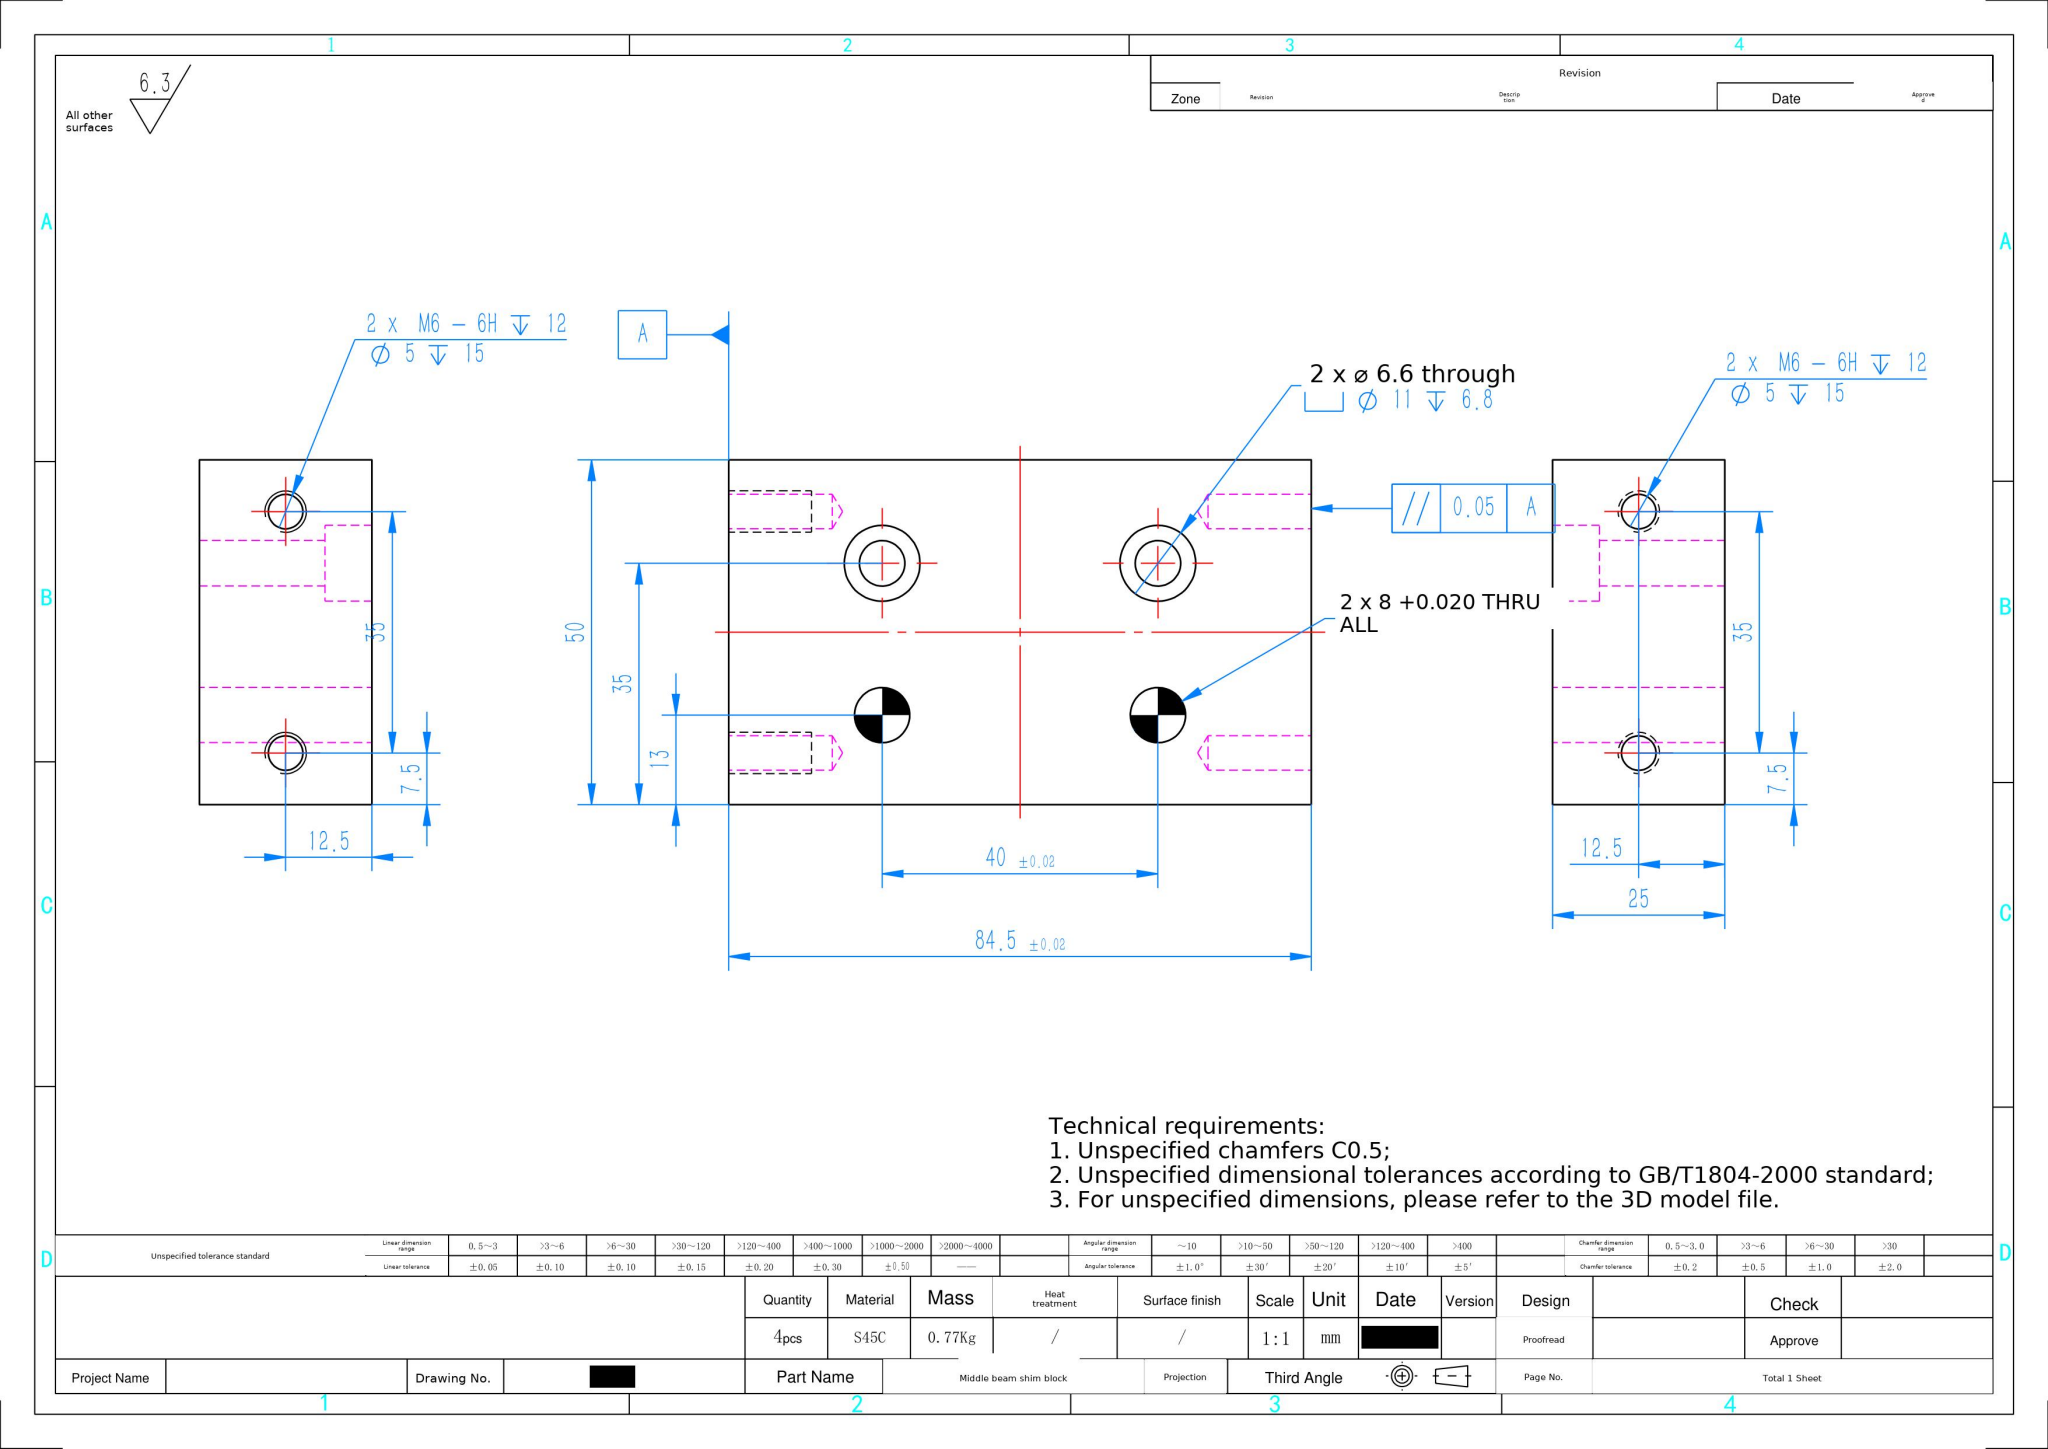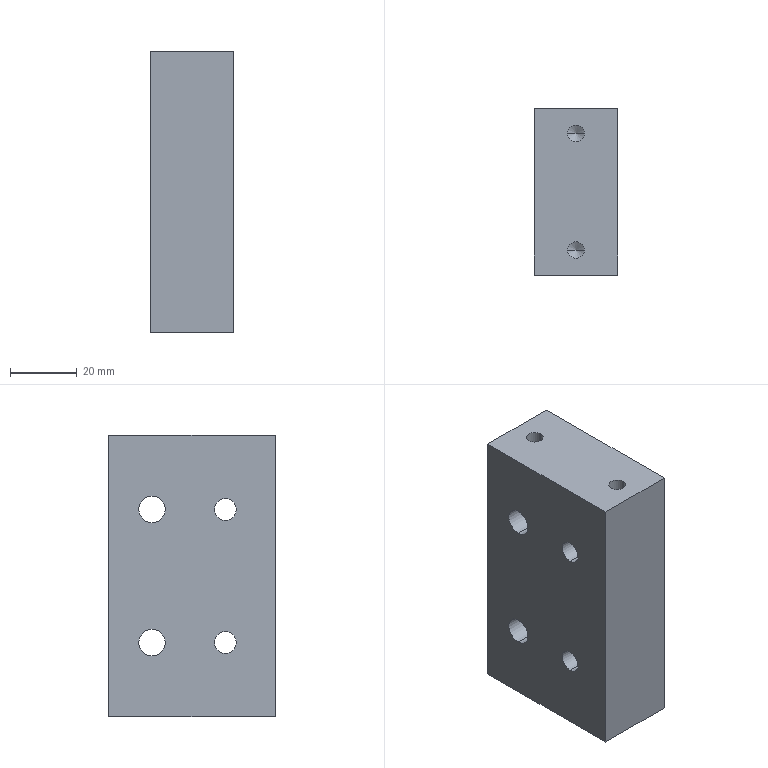Part | SolidWorks | mm | material S45C | 1 solid | 36 faces | box 25 x 50 x 84.5 mm | volume 99357 mm3 | cylinder 20 | cone 8 | plane 8 | commonest cylinder face diameters 5 x8 8 x4 11 x4 6.6 x4
STEP:
#1=CARTESIAN_POINT('',(10.,-17.5,27.25));
#2=VERTEX_POINT('',#1);
#3=CARTESIAN_POINT('',(15.,-17.5,27.25));
#4=VERTEX_POINT('',#3);
#5=CARTESIAN_POINT('',(12.5,-17.5,27.25));
#6=DIRECTION('',(0.,0.,1.));
#7=DIRECTION('',(1.,0.,0.));
#8=AXIS2_PLACEMENT_3D('',#5,#6,#7);
#9=CIRCLE('',#8,2.5);
#10=EDGE_CURVE('',#2,#4,#9,.T.);
#11=ORIENTED_EDGE('',*,*,#10,.F.);
#12=CARTESIAN_POINT('',(10.,-17.5,42.25));
#13=VERTEX_POINT('',#12);
#14=CARTESIAN_POINT('',(10.,-17.5,42.25));
#15=DIRECTION('',(0.,0.,1.));
#16=VECTOR('',#15,1000.);
#17=LINE('',#14,#16);
#18=EDGE_CURVE('',#2,#13,#17,.T.);
#19=ORIENTED_EDGE('',*,*,#18,.T.);
#20=CARTESIAN_POINT('',(15.,-17.5,42.25));
#21=VERTEX_POINT('',#20);
#22=CARTESIAN_POINT('',(12.5,-17.5,42.25));
#23=DIRECTION('',(0.,0.,1.));
#24=DIRECTION('',(1.,0.,0.));
#25=AXIS2_PLACEMENT_3D('',#22,#23,#24);
#26=CIRCLE('',#25,2.5);
#27=EDGE_CURVE('',#13,#21,#26,.T.);
#28=ORIENTED_EDGE('',*,*,#27,.T.);
#29=CARTESIAN_POINT('',(15.,-17.5,42.25));
#30=DIRECTION('',(0.,0.,1.));
#31=VECTOR('',#30,1000.);
#32=LINE('',#29,#31);
#33=EDGE_CURVE('',#4,#21,#32,.T.);
#34=ORIENTED_EDGE('',*,*,#33,.F.);
#35=EDGE_LOOP('',(#11,#19,#28,#34));
#36=FACE_OUTER_BOUND('',#35,.T.);
#37=CARTESIAN_POINT('',(12.5,-17.5,42.25));
#38=DIRECTION('',(0.,0.,1.));
#39=DIRECTION('',(1.,0.,0.));
#40=AXIS2_PLACEMENT_3D('',#37,#38,#39);
#41=CYLINDRICAL_SURFACE('',#40,2.5);
#42=ADVANCED_FACE('',(#36),#41,.F.);
#43=CARTESIAN_POINT('',(12.5,-17.5,25.748));
#44=VERTEX_POINT('',#43);
#45=CARTESIAN_POINT('',(15.,-17.5,27.25));
#46=DIRECTION('',(0.8572,0.,0.515));
#47=VECTOR('',#46,1000.);
#48=LINE('',#45,#47);
#49=EDGE_CURVE('',#44,#4,#48,.T.);
#50=ORIENTED_EDGE('',*,*,#49,.F.);
#51=CARTESIAN_POINT('',(10.,-17.5,27.25));
#52=DIRECTION('',(-0.8572,0.,0.515));
#53=VECTOR('',#52,1000.);
#54=LINE('',#51,#53);
#55=EDGE_CURVE('',#44,#2,#54,.T.);
#56=ORIENTED_EDGE('',*,*,#55,.T.);
#57=ORIENTED_EDGE('',*,*,#10,.T.);
#58=EDGE_LOOP('',(#50,#56,#57));
#59=FACE_OUTER_BOUND('',#58,.T.);
#60=CARTESIAN_POINT('',(12.5,-17.5,27.25));
#61=DIRECTION('',(0.,0.,1.));
#62=DIRECTION('',(1.,0.,0.));
#63=AXIS2_PLACEMENT_3D('',#60,#61,#62);
#64=CONICAL_SURFACE('',#63,2.5,1.03);
#65=ADVANCED_FACE('',(#59),#64,.F.);
#66=CARTESIAN_POINT('',(10.,17.5,27.25));
#67=VERTEX_POINT('',#66);
#68=CARTESIAN_POINT('',(15.,17.5,27.25));
#69=VERTEX_POINT('',#68);
#70=CARTESIAN_POINT('',(12.5,17.5,27.25));
#71=DIRECTION('',(0.,0.,1.));
#72=DIRECTION('',(1.,0.,0.));
#73=AXIS2_PLACEMENT_3D('',#70,#71,#72);
#74=CIRCLE('',#73,2.5);
#75=EDGE_CURVE('',#67,#69,#74,.T.);
#76=ORIENTED_EDGE('',*,*,#75,.F.);
#77=CARTESIAN_POINT('',(10.,17.5,42.25));
#78=VERTEX_POINT('',#77);
#79=CARTESIAN_POINT('',(10.,17.5,42.25));
#80=DIRECTION('',(0.,0.,1.));
#81=VECTOR('',#80,1000.);
#82=LINE('',#79,#81);
#83=EDGE_CURVE('',#67,#78,#82,.T.);
#84=ORIENTED_EDGE('',*,*,#83,.T.);
#85=CARTESIAN_POINT('',(15.,17.5,42.25));
#86=VERTEX_POINT('',#85);
#87=CARTESIAN_POINT('',(12.5,17.5,42.25));
#88=DIRECTION('',(0.,0.,1.));
#89=DIRECTION('',(1.,0.,0.));
#90=AXIS2_PLACEMENT_3D('',#87,#88,#89);
#91=CIRCLE('',#90,2.5);
#92=EDGE_CURVE('',#78,#86,#91,.T.);
#93=ORIENTED_EDGE('',*,*,#92,.T.);
#94=CARTESIAN_POINT('',(15.,17.5,42.25));
#95=DIRECTION('',(0.,0.,1.));
#96=VECTOR('',#95,1000.);
#97=LINE('',#94,#96);
#98=EDGE_CURVE('',#69,#86,#97,.T.);
#99=ORIENTED_EDGE('',*,*,#98,.F.);
#100=EDGE_LOOP('',(#76,#84,#93,#99));
#101=FACE_OUTER_BOUND('',#100,.T.);
#102=CARTESIAN_POINT('',(12.5,17.5,42.25));
#103=DIRECTION('',(0.,0.,1.));
#104=DIRECTION('',(1.,0.,0.));
#105=AXIS2_PLACEMENT_3D('',#102,#103,#104);
#106=CYLINDRICAL_SURFACE('',#105,2.5);
#107=ADVANCED_FACE('',(#101),#106,.F.);
#108=CARTESIAN_POINT('',(12.5,17.5,25.748));
#109=VERTEX_POINT('',#108);
#110=CARTESIAN_POINT('',(15.,17.5,27.25));
#111=DIRECTION('',(0.8572,0.,0.515));
#112=VECTOR('',#111,1000.);
#113=LINE('',#110,#112);
#114=EDGE_CURVE('',#109,#69,#113,.T.);
#115=ORIENTED_EDGE('',*,*,#114,.F.);
#116=CARTESIAN_POINT('',(10.,17.5,27.25));
#117=DIRECTION('',(-0.8572,0.,0.515));
#118=VECTOR('',#117,1000.);
#119=LINE('',#116,#118);
#120=EDGE_CURVE('',#109,#67,#119,.T.);
#121=ORIENTED_EDGE('',*,*,#120,.T.);
#122=ORIENTED_EDGE('',*,*,#75,.T.);
#123=EDGE_LOOP('',(#115,#121,#122));
#124=FACE_OUTER_BOUND('',#123,.T.);
#125=CARTESIAN_POINT('',(12.5,17.5,27.25));
#126=DIRECTION('',(0.,0.,1.));
#127=DIRECTION('',(1.,0.,0.));
#128=AXIS2_PLACEMENT_3D('',#125,#126,#127);
#129=CONICAL_SURFACE('',#128,2.5,1.03);
#130=ADVANCED_FACE('',(#124),#129,.F.);
#131=CARTESIAN_POINT('',(15.,17.5,-27.25));
#132=VERTEX_POINT('',#131);
#133=CARTESIAN_POINT('',(10.,17.5,-27.25));
#134=VERTEX_POINT('',#133);
#135=CARTESIAN_POINT('',(12.5,17.5,-27.25));
#136=DIRECTION('',(0.,0.,-1.));
#137=DIRECTION('',(-1.,0.,0.));
#138=AXIS2_PLACEMENT_3D('',#135,#136,#137);
#139=CIRCLE('',#138,2.5);
#140=EDGE_CURVE('',#132,#134,#139,.T.);
#141=ORIENTED_EDGE('',*,*,#140,.F.);
#142=CARTESIAN_POINT('',(15.,17.5,-42.25));
#143=VERTEX_POINT('',#142);
#144=CARTESIAN_POINT('',(15.,17.5,-42.25));
#145=DIRECTION('',(0.,0.,-1.));
#146=VECTOR('',#145,1000.);
#147=LINE('',#144,#146);
#148=EDGE_CURVE('',#132,#143,#147,.T.);
#149=ORIENTED_EDGE('',*,*,#148,.T.);
#150=CARTESIAN_POINT('',(10.,17.5,-42.25));
#151=VERTEX_POINT('',#150);
#152=CARTESIAN_POINT('',(12.5,17.5,-42.25));
#153=DIRECTION('',(0.,0.,-1.));
#154=DIRECTION('',(-1.,0.,0.));
#155=AXIS2_PLACEMENT_3D('',#152,#153,#154);
#156=CIRCLE('',#155,2.5);
#157=EDGE_CURVE('',#143,#151,#156,.T.);
#158=ORIENTED_EDGE('',*,*,#157,.T.);
#159=CARTESIAN_POINT('',(10.,17.5,-42.25));
#160=DIRECTION('',(0.,0.,-1.));
#161=VECTOR('',#160,1000.);
#162=LINE('',#159,#161);
#163=EDGE_CURVE('',#134,#151,#162,.T.);
#164=ORIENTED_EDGE('',*,*,#163,.F.);
#165=EDGE_LOOP('',(#141,#149,#158,#164));
#166=FACE_OUTER_BOUND('',#165,.T.);
#167=CARTESIAN_POINT('',(12.5,17.5,-42.25));
#168=DIRECTION('',(0.,0.,-1.));
#169=DIRECTION('',(-1.,0.,0.));
#170=AXIS2_PLACEMENT_3D('',#167,#168,#169);
#171=CYLINDRICAL_SURFACE('',#170,2.5);
#172=ADVANCED_FACE('',(#166),#171,.F.);
#173=CARTESIAN_POINT('',(12.5,17.5,-25.748));
#174=VERTEX_POINT('',#173);
#175=CARTESIAN_POINT('',(10.,17.5,-27.25));
#176=DIRECTION('',(-0.8572,0.,-0.515));
#177=VECTOR('',#176,1000.);
#178=LINE('',#175,#177);
#179=EDGE_CURVE('',#174,#134,#178,.T.);
#180=ORIENTED_EDGE('',*,*,#179,.F.);
#181=CARTESIAN_POINT('',(15.,17.5,-27.25));
#182=DIRECTION('',(0.8572,0.,-0.515));
#183=VECTOR('',#182,1000.);
#184=LINE('',#181,#183);
#185=EDGE_CURVE('',#174,#132,#184,.T.);
#186=ORIENTED_EDGE('',*,*,#185,.T.);
#187=ORIENTED_EDGE('',*,*,#140,.T.);
#188=EDGE_LOOP('',(#180,#186,#187));
#189=FACE_OUTER_BOUND('',#188,.T.);
#190=CARTESIAN_POINT('',(12.5,17.5,-27.25));
#191=DIRECTION('',(0.,0.,-1.));
#192=DIRECTION('',(-1.,0.,0.));
#193=AXIS2_PLACEMENT_3D('',#190,#191,#192);
#194=CONICAL_SURFACE('',#193,2.5,1.03);
#195=ADVANCED_FACE('',(#189),#194,.F.);
#196=CARTESIAN_POINT('',(15.,-17.5,-27.25));
#197=VERTEX_POINT('',#196);
#198=CARTESIAN_POINT('',(10.,-17.5,-27.25));
#199=VERTEX_POINT('',#198);
#200=CARTESIAN_POINT('',(12.5,-17.5,-27.25));
#201=DIRECTION('',(0.,0.,-1.));
#202=DIRECTION('',(-1.,0.,0.));
#203=AXIS2_PLACEMENT_3D('',#200,#201,#202);
#204=CIRCLE('',#203,2.5);
#205=EDGE_CURVE('',#197,#199,#204,.T.);
#206=ORIENTED_EDGE('',*,*,#205,.F.);
#207=CARTESIAN_POINT('',(15.,-17.5,-42.25));
#208=VERTEX_POINT('',#207);
#209=CARTESIAN_POINT('',(15.,-17.5,-42.25));
#210=DIRECTION('',(0.,0.,-1.));
#211=VECTOR('',#210,1000.);
#212=LINE('',#209,#211);
#213=EDGE_CURVE('',#197,#208,#212,.T.);
#214=ORIENTED_EDGE('',*,*,#213,.T.);
#215=CARTESIAN_POINT('',(10.,-17.5,-42.25));
#216=VERTEX_POINT('',#215);
#217=CARTESIAN_POINT('',(12.5,-17.5,-42.25));
#218=DIRECTION('',(0.,0.,-1.));
#219=DIRECTION('',(-1.,0.,0.));
#220=AXIS2_PLACEMENT_3D('',#217,#218,#219);
#221=CIRCLE('',#220,2.5);
#222=EDGE_CURVE('',#208,#216,#221,.T.);
#223=ORIENTED_EDGE('',*,*,#222,.T.);
#224=CARTESIAN_POINT('',(10.,-17.5,-42.25));
#225=DIRECTION('',(0.,0.,-1.));
#226=VECTOR('',#225,1000.);
#227=LINE('',#224,#226);
#228=EDGE_CURVE('',#199,#216,#227,.T.);
#229=ORIENTED_EDGE('',*,*,#228,.F.);
#230=EDGE_LOOP('',(#206,#214,#223,#229));
#231=FACE_OUTER_BOUND('',#230,.T.);
#232=CARTESIAN_POINT('',(12.5,-17.5,-42.25));
#233=DIRECTION('',(0.,0.,-1.));
#234=DIRECTION('',(-1.,0.,0.));
#235=AXIS2_PLACEMENT_3D('',#232,#233,#234);
#236=CYLINDRICAL_SURFACE('',#235,2.5);
#237=ADVANCED_FACE('',(#231),#236,.F.);
#238=CARTESIAN_POINT('',(12.5,-17.5,-25.748));
#239=VERTEX_POINT('',#238);
#240=CARTESIAN_POINT('',(10.,-17.5,-27.25));
#241=DIRECTION('',(-0.8572,0.,-0.515));
#242=VECTOR('',#241,1000.);
#243=LINE('',#240,#242);
#244=EDGE_CURVE('',#239,#199,#243,.T.);
#245=ORIENTED_EDGE('',*,*,#244,.F.);
#246=CARTESIAN_POINT('',(15.,-17.5,-27.25));
#247=DIRECTION('',(0.8572,0.,-0.515));
#248=VECTOR('',#247,1000.);
#249=LINE('',#246,#248);
#250=EDGE_CURVE('',#239,#197,#249,.T.);
#251=ORIENTED_EDGE('',*,*,#250,.T.);
#252=ORIENTED_EDGE('',*,*,#205,.T.);
#253=EDGE_LOOP('',(#245,#251,#252));
#254=FACE_OUTER_BOUND('',#253,.T.);
#255=CARTESIAN_POINT('',(12.5,-17.5,-27.25));
#256=DIRECTION('',(0.,0.,-1.));
#257=DIRECTION('',(-1.,0.,0.));
#258=AXIS2_PLACEMENT_3D('',#255,#256,#257);
#259=CONICAL_SURFACE('',#258,2.5,1.03);
#260=ADVANCED_FACE('',(#254),#259,.F.);
#261=CARTESIAN_POINT('',(0.,12.,-16.));
#262=VERTEX_POINT('',#261);
#263=CARTESIAN_POINT('',(0.,12.,-24.));
#264=VERTEX_POINT('',#263);
#265=CARTESIAN_POINT('',(0.,12.,-20.));
#266=DIRECTION('',(1.,0.,0.));
#267=DIRECTION('',(0.,0.,-1.));
#268=AXIS2_PLACEMENT_3D('',#265,#266,#267);
#269=CIRCLE('',#268,4.);
#270=EDGE_CURVE('',#262,#264,#269,.T.);
#271=ORIENTED_EDGE('',*,*,#270,.F.);
#272=CARTESIAN_POINT('',(25.,12.,-16.));
#273=VERTEX_POINT('',#272);
#274=CARTESIAN_POINT('',(25.,12.,-16.));
#275=DIRECTION('',(1.,0.,0.));
#276=VECTOR('',#275,1000.);
#277=LINE('',#274,#276);
#278=EDGE_CURVE('',#262,#273,#277,.T.);
#279=ORIENTED_EDGE('',*,*,#278,.T.);
#280=CARTESIAN_POINT('',(25.,12.,-24.));
#281=VERTEX_POINT('',#280);
#282=CARTESIAN_POINT('',(25.,12.,-20.));
#283=DIRECTION('',(1.,0.,0.));
#284=DIRECTION('',(0.,0.,-1.));
#285=AXIS2_PLACEMENT_3D('',#282,#283,#284);
#286=CIRCLE('',#285,4.);
#287=EDGE_CURVE('',#273,#281,#286,.T.);
#288=ORIENTED_EDGE('',*,*,#287,.T.);
#289=CARTESIAN_POINT('',(25.,12.,-24.));
#290=DIRECTION('',(1.,0.,0.));
#291=VECTOR('',#290,1000.);
#292=LINE('',#289,#291);
#293=EDGE_CURVE('',#264,#281,#292,.T.);
#294=ORIENTED_EDGE('',*,*,#293,.F.);
#295=EDGE_LOOP('',(#271,#279,#288,#294));
#296=FACE_OUTER_BOUND('',#295,.T.);
#297=CARTESIAN_POINT('',(25.,12.,-20.));
#298=DIRECTION('',(1.,0.,0.));
#299=DIRECTION('',(0.,0.,-1.));
#300=AXIS2_PLACEMENT_3D('',#297,#298,#299);
#301=CYLINDRICAL_SURFACE('',#300,4.);
#302=ADVANCED_FACE('',(#296),#301,.F.);
#303=CARTESIAN_POINT('',(0.,12.,24.));
#304=VERTEX_POINT('',#303);
#305=CARTESIAN_POINT('',(0.,12.,16.));
#306=VERTEX_POINT('',#305);
#307=CARTESIAN_POINT('',(0.,12.,20.));
#308=DIRECTION('',(1.,0.,0.));
#309=DIRECTION('',(0.,0.,-1.));
#310=AXIS2_PLACEMENT_3D('',#307,#308,#309);
#311=CIRCLE('',#310,4.);
#312=EDGE_CURVE('',#304,#306,#311,.T.);
#313=ORIENTED_EDGE('',*,*,#312,.F.);
#314=CARTESIAN_POINT('',(25.,12.,24.));
#315=VERTEX_POINT('',#314);
#316=CARTESIAN_POINT('',(25.,12.,24.));
#317=DIRECTION('',(1.,0.,0.));
#318=VECTOR('',#317,1000.);
#319=LINE('',#316,#318);
#320=EDGE_CURVE('',#304,#315,#319,.T.);
#321=ORIENTED_EDGE('',*,*,#320,.T.);
#322=CARTESIAN_POINT('',(25.,12.,16.));
#323=VERTEX_POINT('',#322);
#324=CARTESIAN_POINT('',(25.,12.,20.));
#325=DIRECTION('',(1.,0.,0.));
#326=DIRECTION('',(0.,0.,-1.));
#327=AXIS2_PLACEMENT_3D('',#324,#325,#326);
#328=CIRCLE('',#327,4.);
#329=EDGE_CURVE('',#315,#323,#328,.T.);
#330=ORIENTED_EDGE('',*,*,#329,.T.);
#331=CARTESIAN_POINT('',(25.,12.,16.));
#332=DIRECTION('',(1.,0.,0.));
#333=VECTOR('',#332,1000.);
#334=LINE('',#331,#333);
#335=EDGE_CURVE('',#306,#323,#334,.T.);
#336=ORIENTED_EDGE('',*,*,#335,.F.);
#337=EDGE_LOOP('',(#313,#321,#330,#336));
#338=FACE_OUTER_BOUND('',#337,.T.);
#339=CARTESIAN_POINT('',(25.,12.,20.));
#340=DIRECTION('',(1.,0.,0.));
#341=DIRECTION('',(0.,0.,-1.));
#342=AXIS2_PLACEMENT_3D('',#339,#340,#341);
#343=CYLINDRICAL_SURFACE('',#342,4.);
#344=ADVANCED_FACE('',(#338),#343,.F.);
#345=CARTESIAN_POINT('',(18.2,-10.,-14.5));
#346=VERTEX_POINT('',#345);
#347=CARTESIAN_POINT('',(18.2,-10.,-25.5));
#348=VERTEX_POINT('',#347);
#349=CARTESIAN_POINT('',(18.2,-10.,-20.));
#350=DIRECTION('',(1.,0.,0.));
#351=DIRECTION('',(0.,0.,-1.));
#352=AXIS2_PLACEMENT_3D('',#349,#350,#351);
#353=CIRCLE('',#352,5.5);
#354=EDGE_CURVE('',#346,#348,#353,.T.);
#355=ORIENTED_EDGE('',*,*,#354,.F.);
#356=CARTESIAN_POINT('',(25.,-10.,-14.5));
#357=VERTEX_POINT('',#356);
#358=CARTESIAN_POINT('',(25.,-10.,-14.5));
#359=DIRECTION('',(1.,0.,0.));
#360=VECTOR('',#359,1000.);
#361=LINE('',#358,#360);
#362=EDGE_CURVE('',#346,#357,#361,.T.);
#363=ORIENTED_EDGE('',*,*,#362,.T.);
#364=CARTESIAN_POINT('',(25.,-10.,-25.5));
#365=VERTEX_POINT('',#364);
#366=CARTESIAN_POINT('',(25.,-10.,-20.));
#367=DIRECTION('',(1.,0.,0.));
#368=DIRECTION('',(0.,0.,-1.));
#369=AXIS2_PLACEMENT_3D('',#366,#367,#368);
#370=CIRCLE('',#369,5.5);
#371=EDGE_CURVE('',#357,#365,#370,.T.);
#372=ORIENTED_EDGE('',*,*,#371,.T.);
#373=CARTESIAN_POINT('',(25.,-10.,-25.5));
#374=DIRECTION('',(1.,0.,0.));
#375=VECTOR('',#374,1000.);
#376=LINE('',#373,#375);
#377=EDGE_CURVE('',#348,#365,#376,.T.);
#378=ORIENTED_EDGE('',*,*,#377,.F.);
#379=EDGE_LOOP('',(#355,#363,#372,#378));
#380=FACE_OUTER_BOUND('',#379,.T.);
#381=CARTESIAN_POINT('',(25.,-10.,-20.));
#382=DIRECTION('',(1.,0.,0.));
#383=DIRECTION('',(0.,0.,-1.));
#384=AXIS2_PLACEMENT_3D('',#381,#382,#383);
#385=CYLINDRICAL_SURFACE('',#384,5.5);
#386=ADVANCED_FACE('',(#380),#385,.F.);
#387=CARTESIAN_POINT('',(0.,-10.,-16.7));
#388=VERTEX_POINT('',#387);
#389=CARTESIAN_POINT('',(0.,-10.,-23.3));
#390=VERTEX_POINT('',#389);
#391=CARTESIAN_POINT('',(0.,-10.,-20.));
#392=DIRECTION('',(1.,0.,0.));
#393=DIRECTION('',(0.,0.,-1.));
#394=AXIS2_PLACEMENT_3D('',#391,#392,#393);
#395=CIRCLE('',#394,3.3);
#396=EDGE_CURVE('',#388,#390,#395,.T.);
#397=ORIENTED_EDGE('',*,*,#396,.F.);
#398=CARTESIAN_POINT('',(18.2,-10.,-16.7));
#399=VERTEX_POINT('',#398);
#400=CARTESIAN_POINT('',(25.,-10.,-16.7));
#401=DIRECTION('',(1.,0.,0.));
#402=VECTOR('',#401,1000.);
#403=LINE('',#400,#402);
#404=EDGE_CURVE('',#388,#399,#403,.T.);
#405=ORIENTED_EDGE('',*,*,#404,.T.);
#406=CARTESIAN_POINT('',(18.2,-10.,-23.3));
#407=VERTEX_POINT('',#406);
#408=CARTESIAN_POINT('',(18.2,-10.,-20.));
#409=DIRECTION('',(1.,0.,0.));
#410=DIRECTION('',(0.,0.,-1.));
#411=AXIS2_PLACEMENT_3D('',#408,#409,#410);
#412=CIRCLE('',#411,3.3);
#413=EDGE_CURVE('',#399,#407,#412,.T.);
#414=ORIENTED_EDGE('',*,*,#413,.T.);
#415=CARTESIAN_POINT('',(25.,-10.,-23.3));
#416=DIRECTION('',(1.,0.,0.));
#417=VECTOR('',#416,1000.);
#418=LINE('',#415,#417);
#419=EDGE_CURVE('',#390,#407,#418,.T.);
#420=ORIENTED_EDGE('',*,*,#419,.F.);
#421=EDGE_LOOP('',(#397,#405,#414,#420));
#422=FACE_OUTER_BOUND('',#421,.T.);
#423=CARTESIAN_POINT('',(25.,-10.,-20.));
#424=DIRECTION('',(1.,0.,0.));
#425=DIRECTION('',(0.,0.,-1.));
#426=AXIS2_PLACEMENT_3D('',#423,#424,#425);
#427=CYLINDRICAL_SURFACE('',#426,3.3);
#428=ADVANCED_FACE('',(#422),#427,.F.);
#429=CARTESIAN_POINT('',(18.2,-10.,25.5));
#430=VERTEX_POINT('',#429);
#431=CARTESIAN_POINT('',(18.2,-10.,14.5));
#432=VERTEX_POINT('',#431);
#433=CARTESIAN_POINT('',(18.2,-10.,20.));
#434=DIRECTION('',(1.,0.,0.));
#435=DIRECTION('',(0.,0.,-1.));
#436=AXIS2_PLACEMENT_3D('',#433,#434,#435);
#437=CIRCLE('',#436,5.5);
#438=EDGE_CURVE('',#430,#432,#437,.T.);
#439=ORIENTED_EDGE('',*,*,#438,.F.);
#440=CARTESIAN_POINT('',(25.,-10.,25.5));
#441=VERTEX_POINT('',#440);
#442=CARTESIAN_POINT('',(25.,-10.,25.5));
#443=DIRECTION('',(1.,0.,0.));
#444=VECTOR('',#443,1000.);
#445=LINE('',#442,#444);
#446=EDGE_CURVE('',#430,#441,#445,.T.);
#447=ORIENTED_EDGE('',*,*,#446,.T.);
#448=CARTESIAN_POINT('',(25.,-10.,14.5));
#449=VERTEX_POINT('',#448);
#450=CARTESIAN_POINT('',(25.,-10.,20.));
#451=DIRECTION('',(1.,0.,0.));
#452=DIRECTION('',(0.,0.,-1.));
#453=AXIS2_PLACEMENT_3D('',#450,#451,#452);
#454=CIRCLE('',#453,5.5);
#455=EDGE_CURVE('',#441,#449,#454,.T.);
#456=ORIENTED_EDGE('',*,*,#455,.T.);
#457=CARTESIAN_POINT('',(25.,-10.,14.5));
#458=DIRECTION('',(1.,0.,0.));
#459=VECTOR('',#458,1000.);
#460=LINE('',#457,#459);
#461=EDGE_CURVE('',#432,#449,#460,.T.);
#462=ORIENTED_EDGE('',*,*,#461,.F.);
#463=EDGE_LOOP('',(#439,#447,#456,#462));
#464=FACE_OUTER_BOUND('',#463,.T.);
#465=CARTESIAN_POINT('',(25.,-10.,20.));
#466=DIRECTION('',(1.,0.,0.));
#467=DIRECTION('',(0.,0.,-1.));
#468=AXIS2_PLACEMENT_3D('',#465,#466,#467);
#469=CYLINDRICAL_SURFACE('',#468,5.5);
#470=ADVANCED_FACE('',(#464),#469,.F.);
#471=CARTESIAN_POINT('',(0.,-10.,23.3));
#472=VERTEX_POINT('',#471);
#473=CARTESIAN_POINT('',(0.,-10.,16.7));
#474=VERTEX_POINT('',#473);
#475=CARTESIAN_POINT('',(0.,-10.,20.));
#476=DIRECTION('',(1.,0.,0.));
#477=DIRECTION('',(0.,0.,-1.));
#478=AXIS2_PLACEMENT_3D('',#475,#476,#477);
#479=CIRCLE('',#478,3.3);
#480=EDGE_CURVE('',#472,#474,#479,.T.);
#481=ORIENTED_EDGE('',*,*,#480,.F.);
#482=CARTESIAN_POINT('',(18.2,-10.,23.3));
#483=VERTEX_POINT('',#482);
#484=CARTESIAN_POINT('',(25.,-10.,23.3));
#485=DIRECTION('',(1.,0.,0.));
#486=VECTOR('',#485,1000.);
#487=LINE('',#484,#486);
#488=EDGE_CURVE('',#472,#483,#487,.T.);
#489=ORIENTED_EDGE('',*,*,#488,.T.);
#490=CARTESIAN_POINT('',(18.2,-10.,16.7));
#491=VERTEX_POINT('',#490);
#492=CARTESIAN_POINT('',(18.2,-10.,20.));
#493=DIRECTION('',(1.,0.,0.));
#494=DIRECTION('',(0.,0.,-1.));
#495=AXIS2_PLACEMENT_3D('',#492,#493,#494);
#496=CIRCLE('',#495,3.3);
#497=EDGE_CURVE('',#483,#491,#496,.T.);
#498=ORIENTED_EDGE('',*,*,#497,.T.);
#499=CARTESIAN_POINT('',(25.,-10.,16.7));
#500=DIRECTION('',(1.,0.,0.));
#501=VECTOR('',#500,1000.);
#502=LINE('',#499,#501);
#503=EDGE_CURVE('',#474,#491,#502,.T.);
#504=ORIENTED_EDGE('',*,*,#503,.F.);
#505=EDGE_LOOP('',(#481,#489,#498,#504));
#506=FACE_OUTER_BOUND('',#505,.T.);
#507=CARTESIAN_POINT('',(25.,-10.,20.));
#508=DIRECTION('',(1.,0.,0.));
#509=DIRECTION('',(0.,0.,-1.));
#510=AXIS2_PLACEMENT_3D('',#507,#508,#509);
#511=CYLINDRICAL_SURFACE('',#510,3.3);
#512=ADVANCED_FACE('',(#506),#511,.F.);
#513=CARTESIAN_POINT('',(12.5,17.5,-42.25));
#514=DIRECTION('',(0.,0.,-1.));
#515=DIRECTION('',(-1.,0.,0.));
#516=AXIS2_PLACEMENT_3D('',#513,#514,#515);
#517=CIRCLE('',#516,2.5);
#518=EDGE_CURVE('',#151,#143,#517,.T.);
#519=ORIENTED_EDGE('',*,*,#518,.F.);
#520=ORIENTED_EDGE('',*,*,#157,.F.);
#521=EDGE_LOOP('',(#519,#520));
#522=FACE_BOUND('',#521,.T.);
#523=CARTESIAN_POINT('',(12.5,-17.5,-42.25));
#524=DIRECTION('',(0.,0.,-1.));
#525=DIRECTION('',(-1.,0.,0.));
#526=AXIS2_PLACEMENT_3D('',#523,#524,#525);
#527=CIRCLE('',#526,2.5);
#528=EDGE_CURVE('',#216,#208,#527,.T.);
#529=ORIENTED_EDGE('',*,*,#528,.F.);
#530=ORIENTED_EDGE('',*,*,#222,.F.);
#531=EDGE_LOOP('',(#529,#530));
#532=FACE_BOUND('',#531,.T.);
#533=CARTESIAN_POINT('',(0.,-25.,-42.25));
#534=VERTEX_POINT('',#533);
#535=CARTESIAN_POINT('',(0.,25.,-42.25));
#536=VERTEX_POINT('',#535);
#537=CARTESIAN_POINT('',(0.,25.,-42.25));
#538=DIRECTION('',(0.,1.,0.));
#539=VECTOR('',#538,1000.);
#540=LINE('',#537,#539);
#541=EDGE_CURVE('',#534,#536,#540,.T.);
#542=ORIENTED_EDGE('',*,*,#541,.T.);
#543=CARTESIAN_POINT('',(25.,25.,-42.25));
#544=VERTEX_POINT('',#543);
#545=CARTESIAN_POINT('',(25.,25.,-42.25));
#546=DIRECTION('',(-1.,0.,0.));
#547=VECTOR('',#546,1000.);
#548=LINE('',#545,#547);
#549=EDGE_CURVE('',#544,#536,#548,.T.);
#550=ORIENTED_EDGE('',*,*,#549,.F.);
#551=CARTESIAN_POINT('',(25.,-25.,-42.25));
#552=VERTEX_POINT('',#551);
#553=CARTESIAN_POINT('',(25.,25.,-42.25));
#554=DIRECTION('',(0.,1.,0.));
#555=VECTOR('',#554,1000.);
#556=LINE('',#553,#555);
#557=EDGE_CURVE('',#552,#544,#556,.T.);
#558=ORIENTED_EDGE('',*,*,#557,.F.);
#559=CARTESIAN_POINT('',(25.,-25.,-42.25));
#560=DIRECTION('',(-1.,0.,0.));
#561=VECTOR('',#560,1000.);
#562=LINE('',#559,#561);
#563=EDGE_CURVE('',#552,#534,#562,.T.);
#564=ORIENTED_EDGE('',*,*,#563,.T.);
#565=EDGE_LOOP('',(#542,#550,#558,#564));
#566=FACE_OUTER_BOUND('',#565,.T.);
#567=CARTESIAN_POINT('',(25.,25.,-42.25));
#568=DIRECTION('',(0.,0.,1.));
#569=DIRECTION('',(1.,0.,0.));
#570=AXIS2_PLACEMENT_3D('',#567,#568,#569);
#571=PLANE('',#570);
#572=ADVANCED_FACE('',(#522,#532,#566),#571,.F.);
#573=CARTESIAN_POINT('',(0.,25.,42.25));
#574=VERTEX_POINT('',#573);
#575=CARTESIAN_POINT('',(0.,25.,42.25));
#576=DIRECTION('',(0.,0.,1.));
#577=VECTOR('',#576,1000.);
#578=LINE('',#575,#577);
#579=EDGE_CURVE('',#536,#574,#578,.T.);
#580=ORIENTED_EDGE('',*,*,#579,.T.);
#581=CARTESIAN_POINT('',(25.,25.,42.25));
#582=VERTEX_POINT('',#581);
#583=CARTESIAN_POINT('',(25.,25.,42.25));
#584=DIRECTION('',(-1.,0.,0.));
#585=VECTOR('',#584,1000.);
#586=LINE('',#583,#585);
#587=EDGE_CURVE('',#582,#574,#586,.T.);
#588=ORIENTED_EDGE('',*,*,#587,.F.);
#589=CARTESIAN_POINT('',(25.,25.,42.25));
#590=DIRECTION('',(0.,0.,1.));
#591=VECTOR('',#590,1000.);
#592=LINE('',#589,#591);
#593=EDGE_CURVE('',#544,#582,#592,.T.);
#594=ORIENTED_EDGE('',*,*,#593,.F.);
#595=ORIENTED_EDGE('',*,*,#549,.T.);
#596=EDGE_LOOP('',(#580,#588,#594,#595));
#597=FACE_OUTER_BOUND('',#596,.T.);
#598=CARTESIAN_POINT('',(25.,25.,42.25));
#599=DIRECTION('',(0.,-1.,0.));
#600=DIRECTION('',(0.,0.,-1.));
#601=AXIS2_PLACEMENT_3D('',#598,#599,#600);
#602=PLANE('',#601);
#603=ADVANCED_FACE('',(#597),#602,.F.);
#604=CARTESIAN_POINT('',(12.5,-17.5,42.25));
#605=DIRECTION('',(0.,0.,1.));
#606=DIRECTION('',(1.,0.,0.));
#607=AXIS2_PLACEMENT_3D('',#604,#605,#606);
#608=CIRCLE('',#607,2.5);
#609=EDGE_CURVE('',#21,#13,#608,.T.);
#610=ORIENTED_EDGE('',*,*,#609,.F.);
#611=ORIENTED_EDGE('',*,*,#27,.F.);
#612=EDGE_LOOP('',(#610,#611));
#613=FACE_BOUND('',#612,.T.);
#614=CARTESIAN_POINT('',(12.5,17.5,42.25));
#615=DIRECTION('',(0.,0.,1.));
#616=DIRECTION('',(1.,0.,0.));
#617=AXIS2_PLACEMENT_3D('',#614,#615,#616);
#618=CIRCLE('',#617,2.5);
#619=EDGE_CURVE('',#86,#78,#618,.T.);
#620=ORIENTED_EDGE('',*,*,#619,.F.);
#621=ORIENTED_EDGE('',*,*,#92,.F.);
#622=EDGE_LOOP('',(#620,#621));
#623=FACE_BOUND('',#622,.T.);
#624=CARTESIAN_POINT('',(0.,-25.,42.25));
#625=VERTEX_POINT('',#624);
#626=CARTESIAN_POINT('',(0.,25.,42.25));
#627=DIRECTION('',(0.,-1.,-0.));
#628=VECTOR('',#627,1000.);
#629=LINE('',#626,#628);
#630=EDGE_CURVE('',#574,#625,#629,.T.);
#631=ORIENTED_EDGE('',*,*,#630,.T.);
#632=CARTESIAN_POINT('',(25.,-25.,42.25));
#633=VERTEX_POINT('',#632);
#634=CARTESIAN_POINT('',(25.,-25.,42.25));
#635=DIRECTION('',(-1.,0.,0.));
#636=VECTOR('',#635,1000.);
#637=LINE('',#634,#636);
#638=EDGE_CURVE('',#633,#625,#637,.T.);
#639=ORIENTED_EDGE('',*,*,#638,.F.);
#640=CARTESIAN_POINT('',(25.,25.,42.25));
#641=DIRECTION('',(0.,-1.,-0.));
#642=VECTOR('',#641,1000.);
#643=LINE('',#640,#642);
#644=EDGE_CURVE('',#582,#633,#643,.T.);
#645=ORIENTED_EDGE('',*,*,#644,.F.);
#646=ORIENTED_EDGE('',*,*,#587,.T.);
#647=EDGE_LOOP('',(#631,#639,#645,#646));
#648=FACE_OUTER_BOUND('',#647,.T.);
#649=CARTESIAN_POINT('',(25.,25.,42.25));
#650=DIRECTION('',(0.,0.,-1.));
#651=DIRECTION('',(0.,1.,0.));
#652=AXIS2_PLACEMENT_3D('',#649,#650,#651);
#653=PLANE('',#652);
#654=ADVANCED_FACE('',(#613,#623,#648),#653,.F.);
#655=CARTESIAN_POINT('',(0.,-25.,42.25));
#656=DIRECTION('',(0.,0.,-1.));
#657=VECTOR('',#656,1000.);
#658=LINE('',#655,#657);
#659=EDGE_CURVE('',#625,#534,#658,.T.);
#660=ORIENTED_EDGE('',*,*,#659,.T.);
#661=ORIENTED_EDGE('',*,*,#563,.F.);
#662=CARTESIAN_POINT('',(25.,-25.,42.25));
#663=DIRECTION('',(0.,0.,-1.));
#664=VECTOR('',#663,1000.);
#665=LINE('',#662,#664);
#666=EDGE_CURVE('',#633,#552,#665,.T.);
#667=ORIENTED_EDGE('',*,*,#666,.F.);
#668=ORIENTED_EDGE('',*,*,#638,.T.);
#669=EDGE_LOOP('',(#660,#661,#667,#668));
#670=FACE_OUTER_BOUND('',#669,.T.);
#671=CARTESIAN_POINT('',(25.,-25.,42.25));
#672=DIRECTION('',(0.,1.,0.));
#673=DIRECTION('',(0.,0.,1.));
#674=AXIS2_PLACEMENT_3D('',#671,#672,#673);
#675=PLANE('',#674);
#676=ADVANCED_FACE('',(#670),#675,.F.);
#677=CARTESIAN_POINT('',(25.,12.,-20.));
#678=DIRECTION('',(1.,0.,0.));
#679=DIRECTION('',(0.,0.,-1.));
#680=AXIS2_PLACEMENT_3D('',#677,#678,#679);
#681=CIRCLE('',#680,4.);
#682=EDGE_CURVE('',#281,#273,#681,.T.);
#683=ORIENTED_EDGE('',*,*,#682,.F.);
#684=ORIENTED_EDGE('',*,*,#287,.F.);
#685=EDGE_LOOP('',(#683,#684));
#686=FACE_BOUND('',#685,.T.);
#687=CARTESIAN_POINT('',(25.,12.,20.));
#688=DIRECTION('',(1.,0.,0.));
#689=DIRECTION('',(0.,0.,-1.));
#690=AXIS2_PLACEMENT_3D('',#687,#688,#689);
#691=CIRCLE('',#690,4.);
#692=EDGE_CURVE('',#323,#315,#691,.T.);
#693=ORIENTED_EDGE('',*,*,#692,.F.);
#694=ORIENTED_EDGE('',*,*,#329,.F.);
#695=EDGE_LOOP('',(#693,#694));
#696=FACE_BOUND('',#695,.T.);
#697=CARTESIAN_POINT('',(25.,-10.,-20.));
#698=DIRECTION('',(1.,0.,0.));
#699=DIRECTION('',(0.,0.,-1.));
#700=AXIS2_PLACEMENT_3D('',#697,#698,#699);
#701=CIRCLE('',#700,5.5);
#702=EDGE_CURVE('',#365,#357,#701,.T.);
#703=ORIENTED_EDGE('',*,*,#702,.F.);
#704=ORIENTED_EDGE('',*,*,#371,.F.);
#705=EDGE_LOOP('',(#703,#704));
#706=FACE_BOUND('',#705,.T.);
#707=CARTESIAN_POINT('',(25.,-10.,20.));
#708=DIRECTION('',(1.,0.,0.));
#709=DIRECTION('',(0.,0.,-1.));
#710=AXIS2_PLACEMENT_3D('',#707,#708,#709);
#711=CIRCLE('',#710,5.5);
#712=EDGE_CURVE('',#449,#441,#711,.T.);
#713=ORIENTED_EDGE('',*,*,#712,.F.);
#714=ORIENTED_EDGE('',*,*,#455,.F.);
#715=EDGE_LOOP('',(#713,#714));
#716=FACE_BOUND('',#715,.T.);
#717=ORIENTED_EDGE('',*,*,#557,.T.);
#718=ORIENTED_EDGE('',*,*,#593,.T.);
#719=ORIENTED_EDGE('',*,*,#644,.T.);
#720=ORIENTED_EDGE('',*,*,#666,.T.);
#721=EDGE_LOOP('',(#717,#718,#719,#720));
#722=FACE_OUTER_BOUND('',#721,.T.);
#723=CARTESIAN_POINT('',(25.,0.,0.));
#724=DIRECTION('',(1.,0.,0.));
#725=DIRECTION('',(0.,0.,-1.));
#726=AXIS2_PLACEMENT_3D('',#723,#724,#725);
#727=PLANE('',#726);
#728=ADVANCED_FACE('',(#686,#696,#706,#716,#722),#727,.T.);
#729=CARTESIAN_POINT('',(0.,12.,-20.));
#730=DIRECTION('',(1.,0.,0.));
#731=DIRECTION('',(0.,0.,-1.));
#732=AXIS2_PLACEMENT_3D('',#729,#730,#731);
#733=CIRCLE('',#732,4.);
#734=EDGE_CURVE('',#264,#262,#733,.T.);
#735=ORIENTED_EDGE('',*,*,#734,.T.);
#736=ORIENTED_EDGE('',*,*,#270,.T.);
#737=EDGE_LOOP('',(#735,#736));
#738=FACE_BOUND('',#737,.T.);
#739=CARTESIAN_POINT('',(0.,12.,20.));
#740=DIRECTION('',(1.,0.,0.));
#741=DIRECTION('',(0.,0.,-1.));
#742=AXIS2_PLACEMENT_3D('',#739,#740,#741);
#743=CIRCLE('',#742,4.);
#744=EDGE_CURVE('',#306,#304,#743,.T.);
#745=ORIENTED_EDGE('',*,*,#744,.T.);
#746=ORIENTED_EDGE('',*,*,#312,.T.);
#747=EDGE_LOOP('',(#745,#746));
#748=FACE_BOUND('',#747,.T.);
#749=CARTESIAN_POINT('',(0.,-10.,-20.));
#750=DIRECTION('',(1.,0.,0.));
#751=DIRECTION('',(0.,0.,-1.));
#752=AXIS2_PLACEMENT_3D('',#749,#750,#751);
#753=CIRCLE('',#752,3.3);
#754=EDGE_CURVE('',#390,#388,#753,.T.);
#755=ORIENTED_EDGE('',*,*,#754,.T.);
#756=ORIENTED_EDGE('',*,*,#396,.T.);
#757=EDGE_LOOP('',(#755,#756));
#758=FACE_BOUND('',#757,.T.);
#759=CARTESIAN_POINT('',(0.,-10.,20.));
#760=DIRECTION('',(1.,0.,0.));
#761=DIRECTION('',(0.,0.,-1.));
#762=AXIS2_PLACEMENT_3D('',#759,#760,#761);
#763=CIRCLE('',#762,3.3);
#764=EDGE_CURVE('',#474,#472,#763,.T.);
#765=ORIENTED_EDGE('',*,*,#764,.T.);
#766=ORIENTED_EDGE('',*,*,#480,.T.);
#767=EDGE_LOOP('',(#765,#766));
#768=FACE_BOUND('',#767,.T.);
#769=ORIENTED_EDGE('',*,*,#541,.F.);
#770=ORIENTED_EDGE('',*,*,#659,.F.);
#771=ORIENTED_EDGE('',*,*,#630,.F.);
#772=ORIENTED_EDGE('',*,*,#579,.F.);
#773=EDGE_LOOP('',(#769,#770,#771,#772));
#774=FACE_OUTER_BOUND('',#773,.T.);
#775=CARTESIAN_POINT('',(0.,0.,0.));
#776=DIRECTION('',(1.,0.,0.));
#777=DIRECTION('',(0.,0.,-1.));
#778=AXIS2_PLACEMENT_3D('',#775,#776,#777);
#779=PLANE('',#778);
#780=ADVANCED_FACE('',(#738,#748,#758,#768,#774),#779,.F.);
#781=ORIENTED_EDGE('',*,*,#488,.F.);
#782=ORIENTED_EDGE('',*,*,#764,.F.);
#783=ORIENTED_EDGE('',*,*,#503,.T.);
#784=CARTESIAN_POINT('',(18.2,-10.,20.));
#785=DIRECTION('',(1.,0.,0.));
#786=DIRECTION('',(0.,0.,-1.));
#787=AXIS2_PLACEMENT_3D('',#784,#785,#786);
#788=CIRCLE('',#787,3.3);
#789=EDGE_CURVE('',#491,#483,#788,.T.);
#790=ORIENTED_EDGE('',*,*,#789,.T.);
#791=EDGE_LOOP('',(#781,#782,#783,#790));
#792=FACE_OUTER_BOUND('',#791,.T.);
#793=CARTESIAN_POINT('',(25.,-10.,20.));
#794=DIRECTION('',(1.,0.,0.));
#795=DIRECTION('',(0.,0.,-1.));
#796=AXIS2_PLACEMENT_3D('',#793,#794,#795);
#797=CYLINDRICAL_SURFACE('',#796,3.3);
#798=ADVANCED_FACE('',(#792),#797,.F.);
#799=ORIENTED_EDGE('',*,*,#789,.F.);
#800=ORIENTED_EDGE('',*,*,#497,.F.);
#801=EDGE_LOOP('',(#799,#800));
#802=FACE_BOUND('',#801,.T.);
#803=CARTESIAN_POINT('',(18.2,-10.,20.));
#804=DIRECTION('',(1.,0.,0.));
#805=DIRECTION('',(0.,0.,-1.));
#806=AXIS2_PLACEMENT_3D('',#803,#804,#805);
#807=CIRCLE('',#806,5.5);
#808=EDGE_CURVE('',#432,#430,#807,.T.);
#809=ORIENTED_EDGE('',*,*,#808,.T.);
#810=ORIENTED_EDGE('',*,*,#438,.T.);
#811=EDGE_LOOP('',(#809,#810));
#812=FACE_OUTER_BOUND('',#811,.T.);
#813=CARTESIAN_POINT('',(18.2,-6.7,20.));
#814=DIRECTION('',(-1.,0.,0.));
#815=DIRECTION('',(0.,0.,1.));
#816=AXIS2_PLACEMENT_3D('',#813,#814,#815);
#817=PLANE('',#816);
#818=ADVANCED_FACE('',(#802,#812),#817,.F.);
#819=ORIENTED_EDGE('',*,*,#446,.F.);
#820=ORIENTED_EDGE('',*,*,#808,.F.);
#821=ORIENTED_EDGE('',*,*,#461,.T.);
#822=ORIENTED_EDGE('',*,*,#712,.T.);
#823=EDGE_LOOP('',(#819,#820,#821,#822));
#824=FACE_OUTER_BOUND('',#823,.T.);
#825=CARTESIAN_POINT('',(25.,-10.,20.));
#826=DIRECTION('',(1.,0.,0.));
#827=DIRECTION('',(0.,0.,-1.));
#828=AXIS2_PLACEMENT_3D('',#825,#826,#827);
#829=CYLINDRICAL_SURFACE('',#828,5.5);
#830=ADVANCED_FACE('',(#824),#829,.F.);
#831=ORIENTED_EDGE('',*,*,#404,.F.);
#832=ORIENTED_EDGE('',*,*,#754,.F.);
#833=ORIENTED_EDGE('',*,*,#419,.T.);
#834=CARTESIAN_POINT('',(18.2,-10.,-20.));
#835=DIRECTION('',(1.,0.,0.));
#836=DIRECTION('',(0.,0.,-1.));
#837=AXIS2_PLACEMENT_3D('',#834,#835,#836);
#838=CIRCLE('',#837,3.3);
#839=EDGE_CURVE('',#407,#399,#838,.T.);
#840=ORIENTED_EDGE('',*,*,#839,.T.);
#841=EDGE_LOOP('',(#831,#832,#833,#840));
#842=FACE_OUTER_BOUND('',#841,.T.);
#843=CARTESIAN_POINT('',(25.,-10.,-20.));
#844=DIRECTION('',(1.,0.,0.));
#845=DIRECTION('',(0.,0.,-1.));
#846=AXIS2_PLACEMENT_3D('',#843,#844,#845);
#847=CYLINDRICAL_SURFACE('',#846,3.3);
#848=ADVANCED_FACE('',(#842),#847,.F.);
#849=ORIENTED_EDGE('',*,*,#839,.F.);
#850=ORIENTED_EDGE('',*,*,#413,.F.);
#851=EDGE_LOOP('',(#849,#850));
#852=FACE_BOUND('',#851,.T.);
#853=CARTESIAN_POINT('',(18.2,-10.,-20.));
#854=DIRECTION('',(1.,0.,0.));
#855=DIRECTION('',(0.,0.,-1.));
#856=AXIS2_PLACEMENT_3D('',#853,#854,#855);
#857=CIRCLE('',#856,5.5);
#858=EDGE_CURVE('',#348,#346,#857,.T.);
#859=ORIENTED_EDGE('',*,*,#858,.T.);
#860=ORIENTED_EDGE('',*,*,#354,.T.);
#861=EDGE_LOOP('',(#859,#860));
#862=FACE_OUTER_BOUND('',#861,.T.);
#863=CARTESIAN_POINT('',(18.2,-6.7,-20.));
#864=DIRECTION('',(-1.,0.,0.));
#865=DIRECTION('',(0.,0.,1.));
#866=AXIS2_PLACEMENT_3D('',#863,#864,#865);
#867=PLANE('',#866);
#868=ADVANCED_FACE('',(#852,#862),#867,.F.);
#869=ORIENTED_EDGE('',*,*,#362,.F.);
#870=ORIENTED_EDGE('',*,*,#858,.F.);
#871=ORIENTED_EDGE('',*,*,#377,.T.);
#872=ORIENTED_EDGE('',*,*,#702,.T.);
#873=EDGE_LOOP('',(#869,#870,#871,#872));
#874=FACE_OUTER_BOUND('',#873,.T.);
#875=CARTESIAN_POINT('',(25.,-10.,-20.));
#876=DIRECTION('',(1.,0.,0.));
#877=DIRECTION('',(0.,0.,-1.));
#878=AXIS2_PLACEMENT_3D('',#875,#876,#877);
#879=CYLINDRICAL_SURFACE('',#878,5.5);
#880=ADVANCED_FACE('',(#874),#879,.F.);
#881=ORIENTED_EDGE('',*,*,#320,.F.);
#882=ORIENTED_EDGE('',*,*,#744,.F.);
#883=ORIENTED_EDGE('',*,*,#335,.T.);
#884=ORIENTED_EDGE('',*,*,#692,.T.);
#885=EDGE_LOOP('',(#881,#882,#883,#884));
#886=FACE_OUTER_BOUND('',#885,.T.);
#887=CARTESIAN_POINT('',(25.,12.,20.));
#888=DIRECTION('',(1.,0.,0.));
#889=DIRECTION('',(0.,0.,-1.));
#890=AXIS2_PLACEMENT_3D('',#887,#888,#889);
#891=CYLINDRICAL_SURFACE('',#890,4.);
#892=ADVANCED_FACE('',(#886),#891,.F.);
#893=ORIENTED_EDGE('',*,*,#278,.F.);
#894=ORIENTED_EDGE('',*,*,#734,.F.);
#895=ORIENTED_EDGE('',*,*,#293,.T.);
#896=ORIENTED_EDGE('',*,*,#682,.T.);
#897=EDGE_LOOP('',(#893,#894,#895,#896));
#898=FACE_OUTER_BOUND('',#897,.T.);
#899=CARTESIAN_POINT('',(25.,12.,-20.));
#900=DIRECTION('',(1.,0.,0.));
#901=DIRECTION('',(0.,0.,-1.));
#902=AXIS2_PLACEMENT_3D('',#899,#900,#901);
#903=CYLINDRICAL_SURFACE('',#902,4.);
#904=ADVANCED_FACE('',(#898),#903,.F.);
#905=ORIENTED_EDGE('',*,*,#250,.F.);
#906=ORIENTED_EDGE('',*,*,#244,.T.);
#907=CARTESIAN_POINT('',(12.5,-17.5,-27.25));
#908=DIRECTION('',(0.,0.,-1.));
#909=DIRECTION('',(-1.,0.,0.));
#910=AXIS2_PLACEMENT_3D('',#907,#908,#909);
#911=CIRCLE('',#910,2.5);
#912=EDGE_CURVE('',#199,#197,#911,.T.);
#913=ORIENTED_EDGE('',*,*,#912,.T.);
#914=EDGE_LOOP('',(#905,#906,#913));
#915=FACE_OUTER_BOUND('',#914,.T.);
#916=CARTESIAN_POINT('',(12.5,-17.5,-27.25));
#917=DIRECTION('',(0.,0.,-1.));
#918=DIRECTION('',(-1.,0.,0.));
#919=AXIS2_PLACEMENT_3D('',#916,#917,#918);
#920=CONICAL_SURFACE('',#919,2.5,1.03);
#921=ADVANCED_FACE('',(#915),#920,.F.);
#922=ORIENTED_EDGE('',*,*,#213,.F.);
#923=ORIENTED_EDGE('',*,*,#912,.F.);
#924=ORIENTED_EDGE('',*,*,#228,.T.);
#925=ORIENTED_EDGE('',*,*,#528,.T.);
#926=EDGE_LOOP('',(#922,#923,#924,#925));
#927=FACE_OUTER_BOUND('',#926,.T.);
#928=CARTESIAN_POINT('',(12.5,-17.5,-42.25));
#929=DIRECTION('',(0.,0.,-1.));
#930=DIRECTION('',(-1.,0.,0.));
#931=AXIS2_PLACEMENT_3D('',#928,#929,#930);
#932=CYLINDRICAL_SURFACE('',#931,2.5);
#933=ADVANCED_FACE('',(#927),#932,.F.);
#934=ORIENTED_EDGE('',*,*,#185,.F.);
#935=ORIENTED_EDGE('',*,*,#179,.T.);
#936=CARTESIAN_POINT('',(12.5,17.5,-27.25));
#937=DIRECTION('',(0.,0.,-1.));
#938=DIRECTION('',(-1.,0.,0.));
#939=AXIS2_PLACEMENT_3D('',#936,#937,#938);
#940=CIRCLE('',#939,2.5);
#941=EDGE_CURVE('',#134,#132,#940,.T.);
#942=ORIENTED_EDGE('',*,*,#941,.T.);
#943=EDGE_LOOP('',(#934,#935,#942));
#944=FACE_OUTER_BOUND('',#943,.T.);
#945=CARTESIAN_POINT('',(12.5,17.5,-27.25));
#946=DIRECTION('',(0.,0.,-1.));
#947=DIRECTION('',(-1.,0.,0.));
#948=AXIS2_PLACEMENT_3D('',#945,#946,#947);
#949=CONICAL_SURFACE('',#948,2.5,1.03);
#950=ADVANCED_FACE('',(#944),#949,.F.);
#951=ORIENTED_EDGE('',*,*,#148,.F.);
#952=ORIENTED_EDGE('',*,*,#941,.F.);
#953=ORIENTED_EDGE('',*,*,#163,.T.);
#954=ORIENTED_EDGE('',*,*,#518,.T.);
#955=EDGE_LOOP('',(#951,#952,#953,#954));
#956=FACE_OUTER_BOUND('',#955,.T.);
#957=CARTESIAN_POINT('',(12.5,17.5,-42.25));
#958=DIRECTION('',(0.,0.,-1.));
#959=DIRECTION('',(-1.,0.,0.));
#960=AXIS2_PLACEMENT_3D('',#957,#958,#959);
#961=CYLINDRICAL_SURFACE('',#960,2.5);
#962=ADVANCED_FACE('',(#956),#961,.F.);
#963=ORIENTED_EDGE('',*,*,#120,.F.);
#964=ORIENTED_EDGE('',*,*,#114,.T.);
#965=CARTESIAN_POINT('',(12.5,17.5,27.25));
#966=DIRECTION('',(0.,0.,1.));
#967=DIRECTION('',(1.,0.,0.));
#968=AXIS2_PLACEMENT_3D('',#965,#966,#967);
#969=CIRCLE('',#968,2.5);
#970=EDGE_CURVE('',#69,#67,#969,.T.);
#971=ORIENTED_EDGE('',*,*,#970,.T.);
#972=EDGE_LOOP('',(#963,#964,#971));
#973=FACE_OUTER_BOUND('',#972,.T.);
#974=CARTESIAN_POINT('',(12.5,17.5,27.25));
#975=DIRECTION('',(0.,0.,1.));
#976=DIRECTION('',(1.,0.,0.));
#977=AXIS2_PLACEMENT_3D('',#974,#975,#976);
#978=CONICAL_SURFACE('',#977,2.5,1.03);
#979=ADVANCED_FACE('',(#973),#978,.F.);
#980=ORIENTED_EDGE('',*,*,#83,.F.);
#981=ORIENTED_EDGE('',*,*,#970,.F.);
#982=ORIENTED_EDGE('',*,*,#98,.T.);
#983=ORIENTED_EDGE('',*,*,#619,.T.);
#984=EDGE_LOOP('',(#980,#981,#982,#983));
#985=FACE_OUTER_BOUND('',#984,.T.);
#986=CARTESIAN_POINT('',(12.5,17.5,42.25));
#987=DIRECTION('',(0.,0.,1.));
#988=DIRECTION('',(1.,0.,0.));
#989=AXIS2_PLACEMENT_3D('',#986,#987,#988);
#990=CYLINDRICAL_SURFACE('',#989,2.5);
#991=ADVANCED_FACE('',(#985),#990,.F.);
#992=ORIENTED_EDGE('',*,*,#55,.F.);
#993=ORIENTED_EDGE('',*,*,#49,.T.);
#994=CARTESIAN_POINT('',(12.5,-17.5,27.25));
#995=DIRECTION('',(0.,0.,1.));
#996=DIRECTION('',(1.,0.,0.));
#997=AXIS2_PLACEMENT_3D('',#994,#995,#996);
#998=CIRCLE('',#997,2.5);
#999=EDGE_CURVE('',#4,#2,#998,.T.);
#1000=ORIENTED_EDGE('',*,*,#999,.T.);
#1001=EDGE_LOOP('',(#992,#993,#1000));
#1002=FACE_OUTER_BOUND('',#1001,.T.);
#1003=CARTESIAN_POINT('',(12.5,-17.5,27.25));
#1004=DIRECTION('',(0.,0.,1.));
#1005=DIRECTION('',(1.,0.,0.));
#1006=AXIS2_PLACEMENT_3D('',#1003,#1004,#1005);
#1007=CONICAL_SURFACE('',#1006,2.5,1.03);
#1008=ADVANCED_FACE('',(#1002),#1007,.F.);
#1009=ORIENTED_EDGE('',*,*,#18,.F.);
#1010=ORIENTED_EDGE('',*,*,#999,.F.);
#1011=ORIENTED_EDGE('',*,*,#33,.T.);
#1012=ORIENTED_EDGE('',*,*,#609,.T.);
#1013=EDGE_LOOP('',(#1009,#1010,#1011,#1012));
#1014=FACE_OUTER_BOUND('',#1013,.T.);
#1015=CARTESIAN_POINT('',(12.5,-17.5,42.25));
#1016=DIRECTION('',(0.,0.,1.));
#1017=DIRECTION('',(1.,0.,0.));
#1018=AXIS2_PLACEMENT_3D('',#1015,#1016,#1017);
#1019=CYLINDRICAL_SURFACE('',#1018,2.5);
#1020=ADVANCED_FACE('',(#1014),#1019,.F.);
#1021=CLOSED_SHELL('',(#42,#65,#107,#130,#172,#195,#237,#260,#302,#344,#386,#428,#470,#512,#572,#603,#654,#676,#728,#780,#798,#818,#830,#848,#868,#880,#892,#904,#921,#933,#950,#962,#979,#991,#1008,#1020));
#1022=MANIFOLD_SOLID_BREP('',#1021);
#1023=CARTESIAN_POINT('',(0.,0.,0.));
#1024=DIRECTION('',(0.,0.,1.));
#1025=DIRECTION('',(1.,0.,0.));
#1026=AXIS2_PLACEMENT_3D('',#1023,#1024,#1025);
#1027=(LENGTH_UNIT()NAMED_UNIT(*)SI_UNIT(.MILLI.,.METRE.));
#1028=UNCERTAINTY_MEASURE_WITH_UNIT(LENGTH_MEASURE(0.00001),#1027,'','');
#1029=(NAMED_UNIT(*)PLANE_ANGLE_UNIT()SI_UNIT($,.RADIAN.));
#1030=(NAMED_UNIT(*)SI_UNIT($,.STERADIAN.)SOLID_ANGLE_UNIT());
#1031=(GEOMETRIC_REPRESENTATION_CONTEXT(3)GLOBAL_UNCERTAINTY_ASSIGNED_CONTEXT((#1028))GLOBAL_UNIT_ASSIGNED_CONTEXT((#1027,#1029,#1030))REPRESENTATION_CONTEXT('',''));
#1032=ADVANCED_BREP_SHAPE_REPRESENTATION('',(#1022,#1026),#1031);